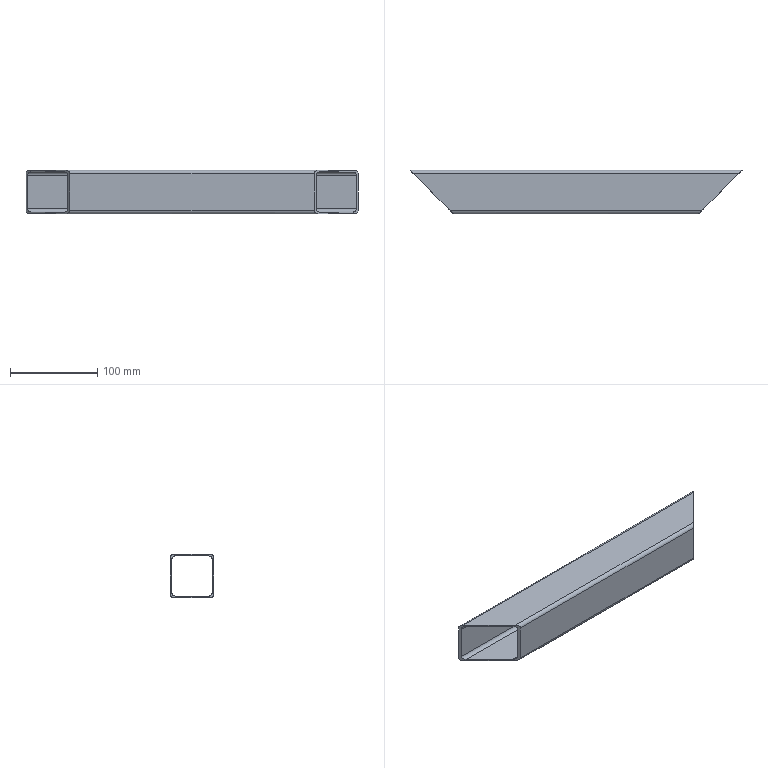Component | NX | SLID_FRAME_BEAM5 | 1 solid | 18 faces | volume 126720 mm3 | plane 10 | cylinder 8 | commonest cylinder face diameters 8 x8